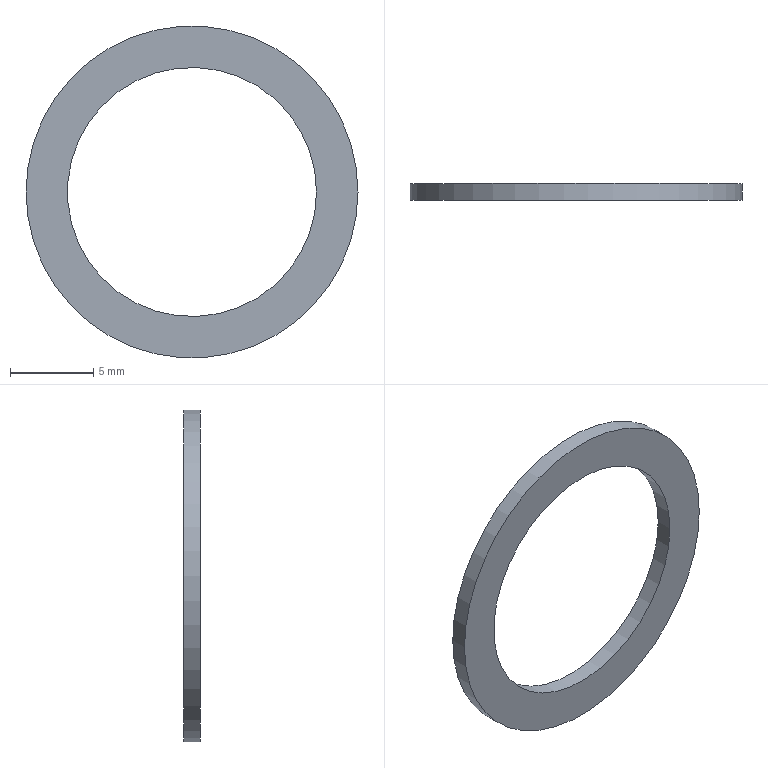Component | NX | SMALL_WASHER_2 | 1 solid | 4 faces | box 20 x 1 x 20 mm | volume 137 mm3 | cylinder 2 | plane 2 | commonest cylinder face diameters 20 x1 15 x1
STEP:
#1=CARTESIAN_POINT('',(0.,0.,0.));
#2=DIRECTION('',(0.,0.,1.));
#3=DIRECTION('',(1.,0.,0.));
#4=AXIS2_PLACEMENT_3D('',#1,#2,#3);
#5=CARTESIAN_POINT('',(26.,39.,-1.));
#6=VERTEX_POINT('',#5);
#7=CARTESIAN_POINT('',(16.,39.,-1.));
#8=DIRECTION('',(0.,-1.,0.));
#9=DIRECTION('',(1.,0.,-0.));
#10=AXIS2_PLACEMENT_3D('',#7,#8,#9);
#11=CIRCLE('',#10,10.);
#12=CARTESIAN_POINT('',(16.,39.,-1.));
#13=DIRECTION('',(0.,-1.,0.));
#14=DIRECTION('',(-1.,0.,0.));
#15=AXIS2_PLACEMENT_3D('',#12,#13,#14);
#16=CYLINDRICAL_SURFACE('',#15,10.);
#17=CARTESIAN_POINT('',(3.142,0.));
#18=DIRECTION('',(1.,0.));
#19=VECTOR('',#18,1.);
#20=LINE('',#17,#19);
#21=(GEOMETRIC_REPRESENTATION_CONTEXT(2)PARAMETRIC_REPRESENTATION_CONTEXT()REPRESENTATION_CONTEXT('',''));
#22=DEFINITIONAL_REPRESENTATION('',(#20),#21);
#23=PCURVE('',#16,#22);
#24=CARTESIAN_POINT('',(16.,39.,-1.));
#25=DIRECTION('',(0.,-1.,0.));
#26=DIRECTION('',(-1.,0.,0.));
#27=AXIS2_PLACEMENT_3D('',#24,#25,#26);
#28=PLANE('',#27);
#29=CARTESIAN_POINT('',(0.,0.));
#30=DIRECTION('',(-1.,0.));
#31=AXIS2_PLACEMENT_2D('',#29,#30);
#32=CIRCLE('',#31,10.);
#33=(GEOMETRIC_REPRESENTATION_CONTEXT(2)PARAMETRIC_REPRESENTATION_CONTEXT()REPRESENTATION_CONTEXT('',''));
#34=DEFINITIONAL_REPRESENTATION('',(#32),#33);
#35=PCURVE('',#28,#34);
#36=SURFACE_CURVE('',#11,(#23,#35),.PCURVE_S1.);
#37=EDGE_CURVE('',#6,#6,#36,.T.);
#38=ORIENTED_EDGE('',*,*,#37,.T.);
#39=CARTESIAN_POINT('',(26.,38.,-1.));
#40=VERTEX_POINT('',#39);
#41=CARTESIAN_POINT('',(26.,39.,-1.));
#42=CARTESIAN_POINT('',(26.,38.,-1.));
#43=B_SPLINE_CURVE_WITH_KNOTS('',1,(#41,#42),.UNSPECIFIED.,.F.,.F.,(2,2),(0.,1.),.PIECEWISE_BEZIER_KNOTS.);
#44=CARTESIAN_POINT('',(9.425,0.));
#45=DIRECTION('',(0.,1.));
#46=VECTOR('',#45,1.);
#47=LINE('',#44,#46);
#48=(GEOMETRIC_REPRESENTATION_CONTEXT(2)PARAMETRIC_REPRESENTATION_CONTEXT()REPRESENTATION_CONTEXT('',''));
#49=DEFINITIONAL_REPRESENTATION('',(#47),#48);
#50=PCURVE('',#16,#49);
#51=CARTESIAN_POINT('',(3.142,0.));
#52=DIRECTION('',(0.,1.));
#53=VECTOR('',#52,1.);
#54=LINE('',#51,#53);
#55=(GEOMETRIC_REPRESENTATION_CONTEXT(2)PARAMETRIC_REPRESENTATION_CONTEXT()REPRESENTATION_CONTEXT('',''));
#56=DEFINITIONAL_REPRESENTATION('',(#54),#55);
#57=PCURVE('',#16,#56);
#58=SEAM_CURVE('',#43,(#50,#57),.PCURVE_S1.);
#59=EDGE_CURVE('',#6,#40,#58,.T.);
#60=ORIENTED_EDGE('',*,*,#59,.T.);
#61=CARTESIAN_POINT('',(16.,38.,-1.));
#62=DIRECTION('',(0.,-1.,0.));
#63=DIRECTION('',(1.,0.,-0.));
#64=AXIS2_PLACEMENT_3D('',#61,#62,#63);
#65=CIRCLE('',#64,10.);
#66=CARTESIAN_POINT('',(3.142,1.));
#67=DIRECTION('',(1.,0.));
#68=VECTOR('',#67,1.);
#69=LINE('',#66,#68);
#70=(GEOMETRIC_REPRESENTATION_CONTEXT(2)PARAMETRIC_REPRESENTATION_CONTEXT()REPRESENTATION_CONTEXT('',''));
#71=DEFINITIONAL_REPRESENTATION('',(#69),#70);
#72=PCURVE('',#16,#71);
#73=CARTESIAN_POINT('',(16.,38.,-1.));
#74=DIRECTION('',(0.,-1.,0.));
#75=DIRECTION('',(-1.,0.,0.));
#76=AXIS2_PLACEMENT_3D('',#73,#74,#75);
#77=PLANE('',#76);
#78=CARTESIAN_POINT('',(0.,0.));
#79=DIRECTION('',(-1.,0.));
#80=AXIS2_PLACEMENT_2D('',#78,#79);
#81=CIRCLE('',#80,10.);
#82=(GEOMETRIC_REPRESENTATION_CONTEXT(2)PARAMETRIC_REPRESENTATION_CONTEXT()REPRESENTATION_CONTEXT('',''));
#83=DEFINITIONAL_REPRESENTATION('',(#81),#82);
#84=PCURVE('',#77,#83);
#85=SURFACE_CURVE('',#65,(#72,#84),.PCURVE_S1.);
#86=EDGE_CURVE('',#40,#40,#85,.T.);
#87=ORIENTED_EDGE('',*,*,#86,.F.);
#88=ORIENTED_EDGE('',*,*,#59,.F.);
#89=EDGE_LOOP('',(#38,#60,#87,#88));
#90=FACE_BOUND('',#89,.T.);
#91=ADVANCED_FACE('',(#90),#16,.T.);
#92=CARTESIAN_POINT('',(23.5,39.,-1.));
#93=VERTEX_POINT('',#92);
#94=CARTESIAN_POINT('',(16.,39.,-1.));
#95=DIRECTION('',(0.,-1.,0.));
#96=DIRECTION('',(1.,0.,-0.));
#97=AXIS2_PLACEMENT_3D('',#94,#95,#96);
#98=CIRCLE('',#97,7.5);
#99=CARTESIAN_POINT('',(16.,39.,-1.));
#100=DIRECTION('',(0.,-1.,0.));
#101=DIRECTION('',(-1.,0.,0.));
#102=AXIS2_PLACEMENT_3D('',#99,#100,#101);
#103=CYLINDRICAL_SURFACE('',#102,7.5);
#104=CARTESIAN_POINT('',(3.142,0.));
#105=DIRECTION('',(1.,0.));
#106=VECTOR('',#105,1.);
#107=LINE('',#104,#106);
#108=(GEOMETRIC_REPRESENTATION_CONTEXT(2)PARAMETRIC_REPRESENTATION_CONTEXT()REPRESENTATION_CONTEXT('',''));
#109=DEFINITIONAL_REPRESENTATION('',(#107),#108);
#110=PCURVE('',#103,#109);
#111=CARTESIAN_POINT('',(0.,0.));
#112=DIRECTION('',(-1.,0.));
#113=AXIS2_PLACEMENT_2D('',#111,#112);
#114=CIRCLE('',#113,7.5);
#115=(GEOMETRIC_REPRESENTATION_CONTEXT(2)PARAMETRIC_REPRESENTATION_CONTEXT()REPRESENTATION_CONTEXT('',''));
#116=DEFINITIONAL_REPRESENTATION('',(#114),#115);
#117=PCURVE('',#28,#116);
#118=SURFACE_CURVE('',#98,(#110,#117),.PCURVE_S1.);
#119=EDGE_CURVE('',#93,#93,#118,.T.);
#120=ORIENTED_EDGE('',*,*,#119,.T.);
#121=CARTESIAN_POINT('',(23.5,38.,-1.));
#122=VERTEX_POINT('',#121);
#123=CARTESIAN_POINT('',(23.5,39.,-1.));
#124=CARTESIAN_POINT('',(23.5,38.,-1.));
#125=B_SPLINE_CURVE_WITH_KNOTS('',1,(#123,#124),.UNSPECIFIED.,.F.,.F.,(2,2),(0.,1.),.PIECEWISE_BEZIER_KNOTS.);
#126=CARTESIAN_POINT('',(9.425,0.));
#127=DIRECTION('',(0.,1.));
#128=VECTOR('',#127,1.);
#129=LINE('',#126,#128);
#130=(GEOMETRIC_REPRESENTATION_CONTEXT(2)PARAMETRIC_REPRESENTATION_CONTEXT()REPRESENTATION_CONTEXT('',''));
#131=DEFINITIONAL_REPRESENTATION('',(#129),#130);
#132=PCURVE('',#103,#131);
#133=CARTESIAN_POINT('',(3.142,0.));
#134=DIRECTION('',(0.,1.));
#135=VECTOR('',#134,1.);
#136=LINE('',#133,#135);
#137=(GEOMETRIC_REPRESENTATION_CONTEXT(2)PARAMETRIC_REPRESENTATION_CONTEXT()REPRESENTATION_CONTEXT('',''));
#138=DEFINITIONAL_REPRESENTATION('',(#136),#137);
#139=PCURVE('',#103,#138);
#140=SEAM_CURVE('',#125,(#132,#139),.PCURVE_S1.);
#141=EDGE_CURVE('',#93,#122,#140,.T.);
#142=ORIENTED_EDGE('',*,*,#141,.T.);
#143=CARTESIAN_POINT('',(16.,38.,-1.));
#144=DIRECTION('',(0.,-1.,0.));
#145=DIRECTION('',(1.,0.,-0.));
#146=AXIS2_PLACEMENT_3D('',#143,#144,#145);
#147=CIRCLE('',#146,7.5);
#148=CARTESIAN_POINT('',(3.142,1.));
#149=DIRECTION('',(1.,0.));
#150=VECTOR('',#149,1.);
#151=LINE('',#148,#150);
#152=(GEOMETRIC_REPRESENTATION_CONTEXT(2)PARAMETRIC_REPRESENTATION_CONTEXT()REPRESENTATION_CONTEXT('',''));
#153=DEFINITIONAL_REPRESENTATION('',(#151),#152);
#154=PCURVE('',#103,#153);
#155=CARTESIAN_POINT('',(0.,0.));
#156=DIRECTION('',(-1.,0.));
#157=AXIS2_PLACEMENT_2D('',#155,#156);
#158=CIRCLE('',#157,7.5);
#159=(GEOMETRIC_REPRESENTATION_CONTEXT(2)PARAMETRIC_REPRESENTATION_CONTEXT()REPRESENTATION_CONTEXT('',''));
#160=DEFINITIONAL_REPRESENTATION('',(#158),#159);
#161=PCURVE('',#77,#160);
#162=SURFACE_CURVE('',#147,(#154,#161),.PCURVE_S1.);
#163=EDGE_CURVE('',#122,#122,#162,.T.);
#164=ORIENTED_EDGE('',*,*,#163,.F.);
#165=ORIENTED_EDGE('',*,*,#141,.F.);
#166=EDGE_LOOP('',(#120,#142,#164,#165));
#167=FACE_BOUND('',#166,.F.);
#168=ADVANCED_FACE('',(#167),#103,.F.);
#169=ORIENTED_EDGE('',*,*,#37,.F.);
#170=EDGE_LOOP('',(#169));
#171=FACE_BOUND('',#170,.T.);
#172=ORIENTED_EDGE('',*,*,#119,.T.);
#173=EDGE_LOOP('',(#172));
#174=FACE_BOUND('',#173,.T.);
#175=ADVANCED_FACE('',(#171,#174),#28,.F.);
#176=ORIENTED_EDGE('',*,*,#86,.T.);
#177=EDGE_LOOP('',(#176));
#178=FACE_BOUND('',#177,.T.);
#179=ORIENTED_EDGE('',*,*,#163,.F.);
#180=EDGE_LOOP('',(#179));
#181=FACE_BOUND('',#180,.T.);
#182=ADVANCED_FACE('',(#178,#181),#77,.T.);
#183=CLOSED_SHELL('',(#91,#168,#175,#182));
#184=MANIFOLD_SOLID_BREP('',#183);
#185=(LENGTH_UNIT()NAMED_UNIT(*)SI_UNIT(.MILLI.,.METRE.));
#186=UNCERTAINTY_MEASURE_WITH_UNIT(LENGTH_MEASURE(0.00001),#185,'','');
#187=(NAMED_UNIT(*)PLANE_ANGLE_UNIT()SI_UNIT($,.RADIAN.));
#188=(NAMED_UNIT(*)SI_UNIT($,.STERADIAN.)SOLID_ANGLE_UNIT());
#189=(GEOMETRIC_REPRESENTATION_CONTEXT(3)GLOBAL_UNCERTAINTY_ASSIGNED_CONTEXT((#186))GLOBAL_UNIT_ASSIGNED_CONTEXT((#185,#187,#188))REPRESENTATION_CONTEXT('',''));
#190=ADVANCED_BREP_SHAPE_REPRESENTATION('',(#4,#184),#189);